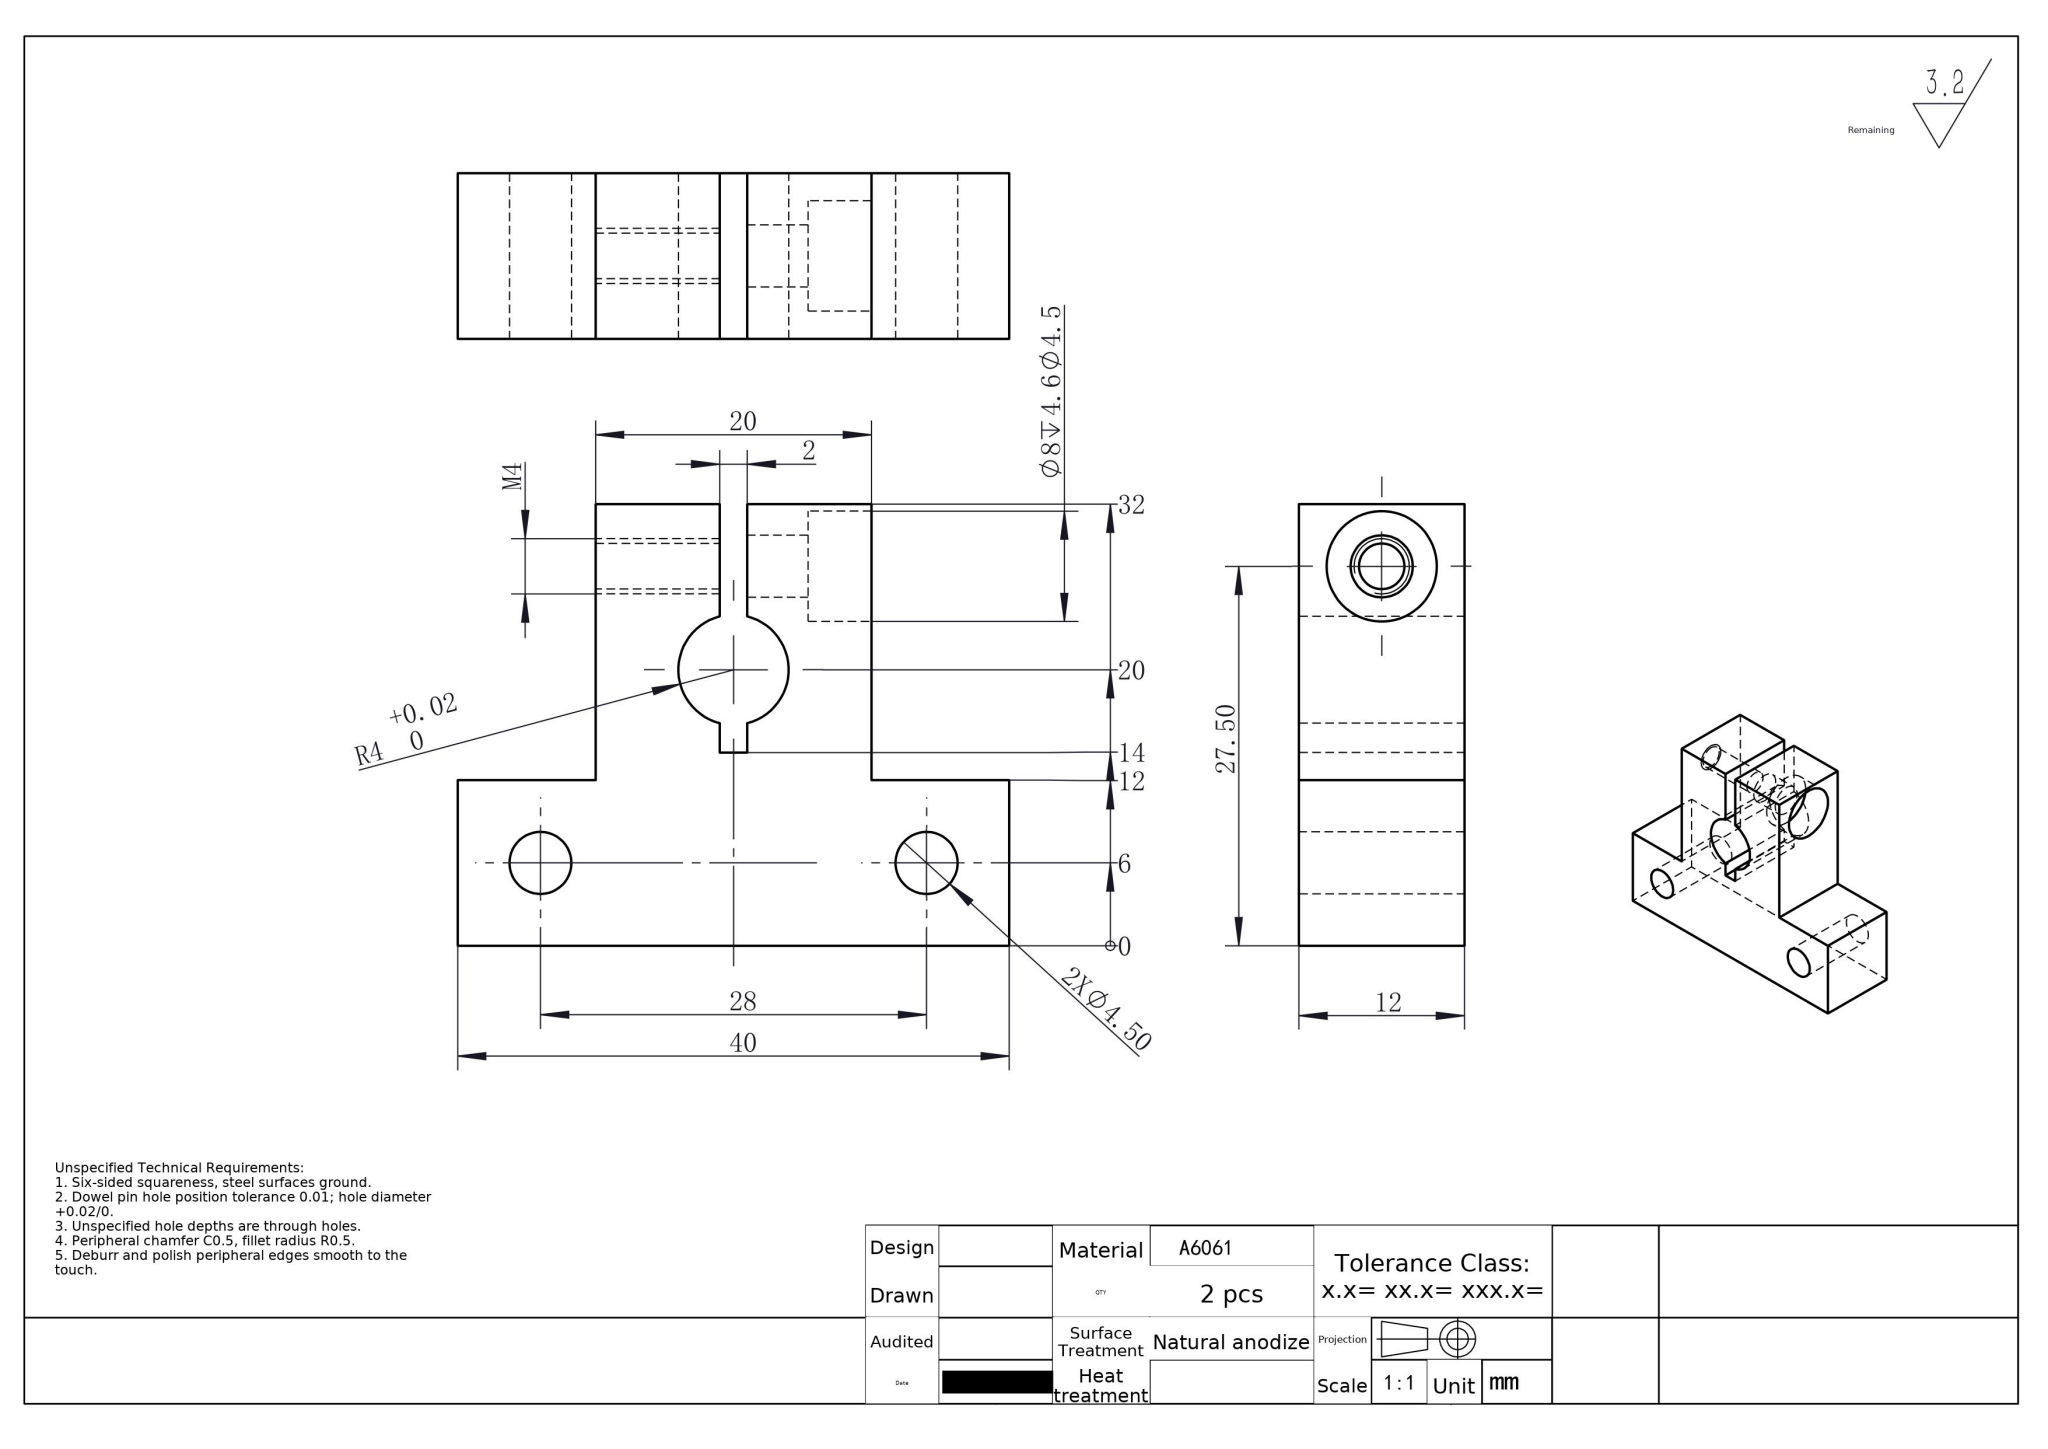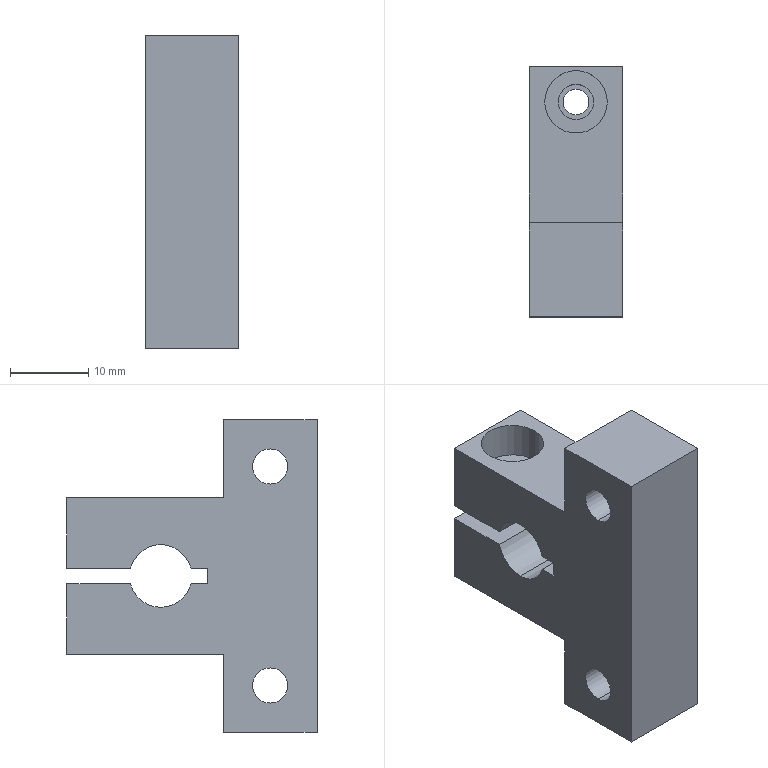Part | NX | mm | 1 solid | 30 faces | box 12 x 32 x 40 mm | volume 8955 mm3 | plane 17 | cylinder 13 | commonest cylinder face diameters 4.5 x6 8 x5 3.3 x2
STEP:
#1=CARTESIAN_POINT('',(0.,25.85,-1.));
#2=VERTEX_POINT('',#1);
#3=CARTESIAN_POINT('',(0.,29.15,-1.));
#4=VERTEX_POINT('',#3);
#5=CARTESIAN_POINT('',(0.,27.5,-1.));
#6=DIRECTION('',(0.,0.,-1.));
#7=DIRECTION('',(-1.,0.,0.));
#8=AXIS2_PLACEMENT_3D('',#5,#6,#7);
#9=CIRCLE('',#8,1.65);
#10=EDGE_CURVE('',#2,#4,#9,.T.);
#11=ORIENTED_EDGE('',*,*,#10,.F.);
#12=CARTESIAN_POINT('',(0.,25.85,-10.));
#13=VERTEX_POINT('',#12);
#14=CARTESIAN_POINT('',(0.,25.85,-10.));
#15=DIRECTION('',(0.,0.,-1.));
#16=VECTOR('',#15,1000.);
#17=LINE('',#14,#16);
#18=EDGE_CURVE('',#2,#13,#17,.T.);
#19=ORIENTED_EDGE('',*,*,#18,.T.);
#20=CARTESIAN_POINT('',(0.,29.15,-10.));
#21=VERTEX_POINT('',#20);
#22=CARTESIAN_POINT('',(0.,27.5,-10.));
#23=DIRECTION('',(0.,0.,-1.));
#24=DIRECTION('',(0.,1.,0.));
#25=AXIS2_PLACEMENT_3D('',#22,#23,#24);
#26=CIRCLE('',#25,1.65);
#27=EDGE_CURVE('',#13,#21,#26,.T.);
#28=ORIENTED_EDGE('',*,*,#27,.T.);
#29=CARTESIAN_POINT('',(0.,29.15,-10.));
#30=DIRECTION('',(0.,0.,-1.));
#31=VECTOR('',#30,1000.);
#32=LINE('',#29,#31);
#33=EDGE_CURVE('',#4,#21,#32,.T.);
#34=ORIENTED_EDGE('',*,*,#33,.F.);
#35=EDGE_LOOP('',(#11,#19,#28,#34));
#36=FACE_OUTER_BOUND('',#35,.T.);
#37=CARTESIAN_POINT('',(0.,27.5,-10.));
#38=DIRECTION('',(0.,0.,-1.));
#39=DIRECTION('',(0.,1.,0.));
#40=AXIS2_PLACEMENT_3D('',#37,#38,#39);
#41=CYLINDRICAL_SURFACE('',#40,1.65);
#42=ADVANCED_FACE('',(#36),#41,.F.);
#43=CARTESIAN_POINT('',(-4.,27.5,5.4));
#44=VERTEX_POINT('',#43);
#45=CARTESIAN_POINT('',(4.,27.5,5.4));
#46=VERTEX_POINT('',#45);
#47=CARTESIAN_POINT('',(0.,27.5,5.4));
#48=DIRECTION('',(0.,0.,1.));
#49=DIRECTION('',(1.,0.,0.));
#50=AXIS2_PLACEMENT_3D('',#47,#48,#49);
#51=CIRCLE('',#50,4.);
#52=EDGE_CURVE('',#44,#46,#51,.T.);
#53=ORIENTED_EDGE('',*,*,#52,.F.);
#54=CARTESIAN_POINT('',(-4.,27.5,10.));
#55=VERTEX_POINT('',#54);
#56=CARTESIAN_POINT('',(-4.,27.5,10.));
#57=DIRECTION('',(0.,0.,1.));
#58=VECTOR('',#57,1000.);
#59=LINE('',#56,#58);
#60=EDGE_CURVE('',#44,#55,#59,.T.);
#61=ORIENTED_EDGE('',*,*,#60,.T.);
#62=CARTESIAN_POINT('',(4.,27.5,10.));
#63=VERTEX_POINT('',#62);
#64=CARTESIAN_POINT('',(0.,27.5,10.));
#65=DIRECTION('',(0.,0.,1.));
#66=DIRECTION('',(1.,0.,0.));
#67=AXIS2_PLACEMENT_3D('',#64,#65,#66);
#68=CIRCLE('',#67,4.);
#69=EDGE_CURVE('',#55,#63,#68,.T.);
#70=ORIENTED_EDGE('',*,*,#69,.T.);
#71=CARTESIAN_POINT('',(4.,27.5,10.));
#72=DIRECTION('',(0.,0.,1.));
#73=VECTOR('',#72,1000.);
#74=LINE('',#71,#73);
#75=EDGE_CURVE('',#46,#63,#74,.T.);
#76=ORIENTED_EDGE('',*,*,#75,.F.);
#77=EDGE_LOOP('',(#53,#61,#70,#76));
#78=FACE_OUTER_BOUND('',#77,.T.);
#79=CARTESIAN_POINT('',(0.,27.5,10.));
#80=DIRECTION('',(0.,0.,1.));
#81=DIRECTION('',(1.,0.,0.));
#82=AXIS2_PLACEMENT_3D('',#79,#80,#81);
#83=CYLINDRICAL_SURFACE('',#82,4.);
#84=ADVANCED_FACE('',(#78),#83,.F.);
#85=CARTESIAN_POINT('',(-2.25,27.5,1.));
#86=VERTEX_POINT('',#85);
#87=CARTESIAN_POINT('',(2.25,27.5,1.));
#88=VERTEX_POINT('',#87);
#89=CARTESIAN_POINT('',(0.,27.5,1.));
#90=DIRECTION('',(0.,-0.,1.));
#91=DIRECTION('',(0.,-1.,-0.));
#92=AXIS2_PLACEMENT_3D('',#89,#90,#91);
#93=CIRCLE('',#92,2.25);
#94=EDGE_CURVE('',#86,#88,#93,.T.);
#95=ORIENTED_EDGE('',*,*,#94,.F.);
#96=CARTESIAN_POINT('',(-2.25,27.5,5.4));
#97=VERTEX_POINT('',#96);
#98=CARTESIAN_POINT('',(-2.25,27.5,10.));
#99=DIRECTION('',(0.,0.,1.));
#100=VECTOR('',#99,1000.);
#101=LINE('',#98,#100);
#102=EDGE_CURVE('',#86,#97,#101,.T.);
#103=ORIENTED_EDGE('',*,*,#102,.T.);
#104=CARTESIAN_POINT('',(2.25,27.5,5.4));
#105=VERTEX_POINT('',#104);
#106=CARTESIAN_POINT('',(0.,27.5,5.4));
#107=DIRECTION('',(0.,0.,1.));
#108=DIRECTION('',(1.,0.,0.));
#109=AXIS2_PLACEMENT_3D('',#106,#107,#108);
#110=CIRCLE('',#109,2.25);
#111=EDGE_CURVE('',#97,#105,#110,.T.);
#112=ORIENTED_EDGE('',*,*,#111,.T.);
#113=CARTESIAN_POINT('',(2.25,27.5,10.));
#114=DIRECTION('',(0.,0.,1.));
#115=VECTOR('',#114,1000.);
#116=LINE('',#113,#115);
#117=EDGE_CURVE('',#88,#105,#116,.T.);
#118=ORIENTED_EDGE('',*,*,#117,.F.);
#119=EDGE_LOOP('',(#95,#103,#112,#118));
#120=FACE_OUTER_BOUND('',#119,.T.);
#121=CARTESIAN_POINT('',(0.,27.5,10.));
#122=DIRECTION('',(0.,0.,1.));
#123=DIRECTION('',(1.,0.,0.));
#124=AXIS2_PLACEMENT_3D('',#121,#122,#123);
#125=CYLINDRICAL_SURFACE('',#124,2.25);
#126=ADVANCED_FACE('',(#120),#125,.F.);
#127=CARTESIAN_POINT('',(-6.,6.,-16.25));
#128=VERTEX_POINT('',#127);
#129=CARTESIAN_POINT('',(-6.,6.,-11.75));
#130=VERTEX_POINT('',#129);
#131=CARTESIAN_POINT('',(-6.,6.,-14.));
#132=DIRECTION('',(-1.,0.,0.));
#133=DIRECTION('',(0.,0.,1.));
#134=AXIS2_PLACEMENT_3D('',#131,#132,#133);
#135=CIRCLE('',#134,2.25);
#136=EDGE_CURVE('',#128,#130,#135,.T.);
#137=ORIENTED_EDGE('',*,*,#136,.T.);
#138=CARTESIAN_POINT('',(6.,6.,-11.75));
#139=VERTEX_POINT('',#138);
#140=CARTESIAN_POINT('',(-14.,6.,-11.75));
#141=DIRECTION('',(1.,0.,0.));
#142=VECTOR('',#141,1000.);
#143=LINE('',#140,#142);
#144=EDGE_CURVE('',#130,#139,#143,.T.);
#145=ORIENTED_EDGE('',*,*,#144,.T.);
#146=CARTESIAN_POINT('',(6.,6.,-16.25));
#147=VERTEX_POINT('',#146);
#148=CARTESIAN_POINT('',(6.,6.,-14.));
#149=DIRECTION('',(1.,0.,0.));
#150=DIRECTION('',(0.,0.,-1.));
#151=AXIS2_PLACEMENT_3D('',#148,#149,#150);
#152=CIRCLE('',#151,2.25);
#153=EDGE_CURVE('',#139,#147,#152,.T.);
#154=ORIENTED_EDGE('',*,*,#153,.T.);
#155=CARTESIAN_POINT('',(-14.,6.,-16.25));
#156=DIRECTION('',(1.,0.,0.));
#157=VECTOR('',#156,1000.);
#158=LINE('',#155,#157);
#159=EDGE_CURVE('',#128,#147,#158,.T.);
#160=ORIENTED_EDGE('',*,*,#159,.F.);
#161=EDGE_LOOP('',(#137,#145,#154,#160));
#162=FACE_OUTER_BOUND('',#161,.T.);
#163=CARTESIAN_POINT('',(-14.,6.,-14.));
#164=DIRECTION('',(1.,0.,0.));
#165=DIRECTION('',(0.,0.,-1.));
#166=AXIS2_PLACEMENT_3D('',#163,#164,#165);
#167=CYLINDRICAL_SURFACE('',#166,2.25);
#168=ADVANCED_FACE('',(#162),#167,.F.);
#169=CARTESIAN_POINT('',(-6.,6.,11.75));
#170=VERTEX_POINT('',#169);
#171=CARTESIAN_POINT('',(-6.,6.,16.25));
#172=VERTEX_POINT('',#171);
#173=CARTESIAN_POINT('',(-6.,6.,14.));
#174=DIRECTION('',(-1.,0.,0.));
#175=DIRECTION('',(0.,0.,1.));
#176=AXIS2_PLACEMENT_3D('',#173,#174,#175);
#177=CIRCLE('',#176,2.25);
#178=EDGE_CURVE('',#170,#172,#177,.T.);
#179=ORIENTED_EDGE('',*,*,#178,.T.);
#180=CARTESIAN_POINT('',(6.,6.,16.25));
#181=VERTEX_POINT('',#180);
#182=CARTESIAN_POINT('',(-14.,6.,16.25));
#183=DIRECTION('',(1.,0.,0.));
#184=VECTOR('',#183,1000.);
#185=LINE('',#182,#184);
#186=EDGE_CURVE('',#172,#181,#185,.T.);
#187=ORIENTED_EDGE('',*,*,#186,.T.);
#188=CARTESIAN_POINT('',(6.,6.,11.75));
#189=VERTEX_POINT('',#188);
#190=CARTESIAN_POINT('',(6.,6.,14.));
#191=DIRECTION('',(1.,0.,0.));
#192=DIRECTION('',(0.,0.,-1.));
#193=AXIS2_PLACEMENT_3D('',#190,#191,#192);
#194=CIRCLE('',#193,2.25);
#195=EDGE_CURVE('',#181,#189,#194,.T.);
#196=ORIENTED_EDGE('',*,*,#195,.T.);
#197=CARTESIAN_POINT('',(-14.,6.,11.75));
#198=DIRECTION('',(1.,0.,0.));
#199=VECTOR('',#198,1000.);
#200=LINE('',#197,#199);
#201=EDGE_CURVE('',#170,#189,#200,.T.);
#202=ORIENTED_EDGE('',*,*,#201,.F.);
#203=EDGE_LOOP('',(#179,#187,#196,#202));
#204=FACE_OUTER_BOUND('',#203,.T.);
#205=CARTESIAN_POINT('',(-14.,6.,14.));
#206=DIRECTION('',(1.,0.,0.));
#207=DIRECTION('',(0.,0.,-1.));
#208=AXIS2_PLACEMENT_3D('',#205,#206,#207);
#209=CYLINDRICAL_SURFACE('',#208,2.25);
#210=ADVANCED_FACE('',(#204),#209,.F.);
#211=CARTESIAN_POINT('',(-6.,23.873,-1.));
#212=VERTEX_POINT('',#211);
#213=CARTESIAN_POINT('',(-6.,20.,-4.));
#214=VERTEX_POINT('',#213);
#215=CARTESIAN_POINT('',(-6.,20.,0.));
#216=DIRECTION('',(-1.,0.,0.));
#217=DIRECTION('',(0.,0.,1.));
#218=AXIS2_PLACEMENT_3D('',#215,#216,#217);
#219=CIRCLE('',#218,4.);
#220=EDGE_CURVE('',#212,#214,#219,.T.);
#221=ORIENTED_EDGE('',*,*,#220,.T.);
#222=CARTESIAN_POINT('',(6.,20.,-4.));
#223=VERTEX_POINT('',#222);
#224=CARTESIAN_POINT('',(-31.,20.,-4.));
#225=DIRECTION('',(1.,0.,0.));
#226=VECTOR('',#225,1000.);
#227=LINE('',#224,#226);
#228=EDGE_CURVE('',#214,#223,#227,.T.);
#229=ORIENTED_EDGE('',*,*,#228,.T.);
#230=CARTESIAN_POINT('',(6.,23.873,-1.));
#231=VERTEX_POINT('',#230);
#232=CARTESIAN_POINT('',(6.,20.,0.));
#233=DIRECTION('',(-1.,0.,0.));
#234=DIRECTION('',(0.,0.,1.));
#235=AXIS2_PLACEMENT_3D('',#232,#233,#234);
#236=CIRCLE('',#235,4.);
#237=EDGE_CURVE('',#231,#223,#236,.T.);
#238=ORIENTED_EDGE('',*,*,#237,.F.);
#239=CARTESIAN_POINT('',(-31.,23.873,-1.));
#240=DIRECTION('',(1.,0.,0.));
#241=VECTOR('',#240,1000.);
#242=LINE('',#239,#241);
#243=EDGE_CURVE('',#212,#231,#242,.T.);
#244=ORIENTED_EDGE('',*,*,#243,.F.);
#245=EDGE_LOOP('',(#221,#229,#238,#244));
#246=FACE_OUTER_BOUND('',#245,.T.);
#247=CARTESIAN_POINT('',(-31.,20.,0.));
#248=DIRECTION('',(1.,0.,0.));
#249=DIRECTION('',(0.,0.,-1.));
#250=AXIS2_PLACEMENT_3D('',#247,#248,#249);
#251=CYLINDRICAL_SURFACE('',#250,4.);
#252=ADVANCED_FACE('',(#246),#251,.F.);
#253=CARTESIAN_POINT('',(-6.,32.,-10.));
#254=VERTEX_POINT('',#253);
#255=CARTESIAN_POINT('',(-6.,32.,-1.));
#256=VERTEX_POINT('',#255);
#257=CARTESIAN_POINT('',(-6.,32.,10.));
#258=DIRECTION('',(0.,0.,1.));
#259=VECTOR('',#258,1000.);
#260=LINE('',#257,#259);
#261=EDGE_CURVE('',#254,#256,#260,.T.);
#262=ORIENTED_EDGE('',*,*,#261,.T.);
#263=CARTESIAN_POINT('',(6.,32.,-1.));
#264=VERTEX_POINT('',#263);
#265=CARTESIAN_POINT('',(-31.,32.,-1.));
#266=DIRECTION('',(1.,0.,0.));
#267=VECTOR('',#266,1000.);
#268=LINE('',#265,#267);
#269=EDGE_CURVE('',#256,#264,#268,.T.);
#270=ORIENTED_EDGE('',*,*,#269,.T.);
#271=CARTESIAN_POINT('',(6.,32.,-10.));
#272=VERTEX_POINT('',#271);
#273=CARTESIAN_POINT('',(6.,32.,10.));
#274=DIRECTION('',(0.,0.,1.));
#275=VECTOR('',#274,1000.);
#276=LINE('',#273,#275);
#277=EDGE_CURVE('',#272,#264,#276,.T.);
#278=ORIENTED_EDGE('',*,*,#277,.F.);
#279=CARTESIAN_POINT('',(6.,32.,-10.));
#280=DIRECTION('',(-1.,0.,0.));
#281=VECTOR('',#280,1000.);
#282=LINE('',#279,#281);
#283=EDGE_CURVE('',#272,#254,#282,.T.);
#284=ORIENTED_EDGE('',*,*,#283,.T.);
#285=EDGE_LOOP('',(#262,#270,#278,#284));
#286=FACE_OUTER_BOUND('',#285,.T.);
#287=CARTESIAN_POINT('',(6.,32.,10.));
#288=DIRECTION('',(0.,-1.,0.));
#289=DIRECTION('',(0.,0.,-1.));
#290=AXIS2_PLACEMENT_3D('',#287,#288,#289);
#291=PLANE('',#290);
#292=ADVANCED_FACE('',(#286),#291,.F.);
#293=CARTESIAN_POINT('',(-6.,12.,20.));
#294=VERTEX_POINT('',#293);
#295=CARTESIAN_POINT('',(-6.,0.,20.));
#296=VERTEX_POINT('',#295);
#297=CARTESIAN_POINT('',(-6.,0.,20.));
#298=DIRECTION('',(0.,-1.,0.));
#299=VECTOR('',#298,1000.);
#300=LINE('',#297,#299);
#301=EDGE_CURVE('',#294,#296,#300,.T.);
#302=ORIENTED_EDGE('',*,*,#301,.T.);
#303=CARTESIAN_POINT('',(6.,0.,20.));
#304=VERTEX_POINT('',#303);
#305=CARTESIAN_POINT('',(6.,0.,20.));
#306=DIRECTION('',(-1.,0.,0.));
#307=VECTOR('',#306,1000.);
#308=LINE('',#305,#307);
#309=EDGE_CURVE('',#304,#296,#308,.T.);
#310=ORIENTED_EDGE('',*,*,#309,.F.);
#311=CARTESIAN_POINT('',(6.,12.,20.));
#312=VERTEX_POINT('',#311);
#313=CARTESIAN_POINT('',(6.,0.,20.));
#314=DIRECTION('',(0.,-1.,0.));
#315=VECTOR('',#314,1000.);
#316=LINE('',#313,#315);
#317=EDGE_CURVE('',#312,#304,#316,.T.);
#318=ORIENTED_EDGE('',*,*,#317,.F.);
#319=CARTESIAN_POINT('',(6.,12.,20.));
#320=DIRECTION('',(-1.,0.,0.));
#321=VECTOR('',#320,1000.);
#322=LINE('',#319,#321);
#323=EDGE_CURVE('',#312,#294,#322,.T.);
#324=ORIENTED_EDGE('',*,*,#323,.T.);
#325=EDGE_LOOP('',(#302,#310,#318,#324));
#326=FACE_OUTER_BOUND('',#325,.T.);
#327=CARTESIAN_POINT('',(6.,0.,20.));
#328=DIRECTION('',(0.,-0.,-1.));
#329=DIRECTION('',(0.,1.,-0.));
#330=AXIS2_PLACEMENT_3D('',#327,#328,#329);
#331=PLANE('',#330);
#332=ADVANCED_FACE('',(#326),#331,.F.);
#333=CARTESIAN_POINT('',(-6.,0.,-20.));
#334=VERTEX_POINT('',#333);
#335=CARTESIAN_POINT('',(-6.,0.,20.));
#336=DIRECTION('',(0.,0.,-1.));
#337=VECTOR('',#336,1000.);
#338=LINE('',#335,#337);
#339=EDGE_CURVE('',#296,#334,#338,.T.);
#340=ORIENTED_EDGE('',*,*,#339,.T.);
#341=CARTESIAN_POINT('',(6.,0.,-20.));
#342=VERTEX_POINT('',#341);
#343=CARTESIAN_POINT('',(6.,0.,-20.));
#344=DIRECTION('',(-1.,0.,0.));
#345=VECTOR('',#344,1000.);
#346=LINE('',#343,#345);
#347=EDGE_CURVE('',#342,#334,#346,.T.);
#348=ORIENTED_EDGE('',*,*,#347,.F.);
#349=CARTESIAN_POINT('',(6.,0.,20.));
#350=DIRECTION('',(0.,0.,-1.));
#351=VECTOR('',#350,1000.);
#352=LINE('',#349,#351);
#353=EDGE_CURVE('',#304,#342,#352,.T.);
#354=ORIENTED_EDGE('',*,*,#353,.F.);
#355=ORIENTED_EDGE('',*,*,#309,.T.);
#356=EDGE_LOOP('',(#340,#348,#354,#355));
#357=FACE_OUTER_BOUND('',#356,.T.);
#358=CARTESIAN_POINT('',(6.,0.,20.));
#359=DIRECTION('',(0.,1.,0.));
#360=DIRECTION('',(0.,0.,1.));
#361=AXIS2_PLACEMENT_3D('',#358,#359,#360);
#362=PLANE('',#361);
#363=ADVANCED_FACE('',(#357),#362,.F.);
#364=CARTESIAN_POINT('',(-6.,12.,-20.));
#365=VERTEX_POINT('',#364);
#366=CARTESIAN_POINT('',(-6.,12.,-20.));
#367=DIRECTION('',(0.,1.,0.));
#368=VECTOR('',#367,1000.);
#369=LINE('',#366,#368);
#370=EDGE_CURVE('',#334,#365,#369,.T.);
#371=ORIENTED_EDGE('',*,*,#370,.T.);
#372=CARTESIAN_POINT('',(6.,12.,-20.));
#373=VERTEX_POINT('',#372);
#374=CARTESIAN_POINT('',(6.,12.,-20.));
#375=DIRECTION('',(-1.,0.,0.));
#376=VECTOR('',#375,1000.);
#377=LINE('',#374,#376);
#378=EDGE_CURVE('',#373,#365,#377,.T.);
#379=ORIENTED_EDGE('',*,*,#378,.F.);
#380=CARTESIAN_POINT('',(6.,12.,-20.));
#381=DIRECTION('',(0.,1.,0.));
#382=VECTOR('',#381,1000.);
#383=LINE('',#380,#382);
#384=EDGE_CURVE('',#342,#373,#383,.T.);
#385=ORIENTED_EDGE('',*,*,#384,.F.);
#386=ORIENTED_EDGE('',*,*,#347,.T.);
#387=EDGE_LOOP('',(#371,#379,#385,#386));
#388=FACE_OUTER_BOUND('',#387,.T.);
#389=CARTESIAN_POINT('',(6.,12.,-20.));
#390=DIRECTION('',(0.,-0.,1.));
#391=DIRECTION('',(0.,-1.,-0.));
#392=AXIS2_PLACEMENT_3D('',#389,#390,#391);
#393=PLANE('',#392);
#394=ADVANCED_FACE('',(#388),#393,.F.);
#395=CARTESIAN_POINT('',(-6.,12.,-10.));
#396=VERTEX_POINT('',#395);
#397=CARTESIAN_POINT('',(-6.,12.,-10.));
#398=DIRECTION('',(0.,0.,1.));
#399=VECTOR('',#398,1000.);
#400=LINE('',#397,#399);
#401=EDGE_CURVE('',#365,#396,#400,.T.);
#402=ORIENTED_EDGE('',*,*,#401,.T.);
#403=CARTESIAN_POINT('',(6.,12.,-10.));
#404=VERTEX_POINT('',#403);
#405=CARTESIAN_POINT('',(6.,12.,-10.));
#406=DIRECTION('',(-1.,0.,0.));
#407=VECTOR('',#406,1000.);
#408=LINE('',#405,#407);
#409=EDGE_CURVE('',#404,#396,#408,.T.);
#410=ORIENTED_EDGE('',*,*,#409,.F.);
#411=CARTESIAN_POINT('',(6.,12.,-10.));
#412=DIRECTION('',(0.,0.,1.));
#413=VECTOR('',#412,1000.);
#414=LINE('',#411,#413);
#415=EDGE_CURVE('',#373,#404,#414,.T.);
#416=ORIENTED_EDGE('',*,*,#415,.F.);
#417=ORIENTED_EDGE('',*,*,#378,.T.);
#418=EDGE_LOOP('',(#402,#410,#416,#417));
#419=FACE_OUTER_BOUND('',#418,.T.);
#420=CARTESIAN_POINT('',(6.,12.,-10.));
#421=DIRECTION('',(0.,-1.,0.));
#422=DIRECTION('',(0.,0.,-1.));
#423=AXIS2_PLACEMENT_3D('',#420,#421,#422);
#424=PLANE('',#423);
#425=ADVANCED_FACE('',(#419),#424,.F.);
#426=CARTESIAN_POINT('',(0.,27.5,-10.));
#427=DIRECTION('',(0.,0.,-1.));
#428=DIRECTION('',(0.,1.,0.));
#429=AXIS2_PLACEMENT_3D('',#426,#427,#428);
#430=CIRCLE('',#429,1.65);
#431=EDGE_CURVE('',#21,#13,#430,.T.);
#432=ORIENTED_EDGE('',*,*,#431,.F.);
#433=ORIENTED_EDGE('',*,*,#27,.F.);
#434=EDGE_LOOP('',(#432,#433));
#435=FACE_BOUND('',#434,.T.);
#436=CARTESIAN_POINT('',(-6.,32.,-10.));
#437=DIRECTION('',(0.,1.,0.));
#438=VECTOR('',#437,1000.);
#439=LINE('',#436,#438);
#440=EDGE_CURVE('',#396,#254,#439,.T.);
#441=ORIENTED_EDGE('',*,*,#440,.T.);
#442=ORIENTED_EDGE('',*,*,#283,.F.);
#443=CARTESIAN_POINT('',(6.,32.,-10.));
#444=DIRECTION('',(0.,1.,0.));
#445=VECTOR('',#444,1000.);
#446=LINE('',#443,#445);
#447=EDGE_CURVE('',#404,#272,#446,.T.);
#448=ORIENTED_EDGE('',*,*,#447,.F.);
#449=ORIENTED_EDGE('',*,*,#409,.T.);
#450=EDGE_LOOP('',(#441,#442,#448,#449));
#451=FACE_OUTER_BOUND('',#450,.T.);
#452=CARTESIAN_POINT('',(6.,32.,-10.));
#453=DIRECTION('',(0.,-0.,1.));
#454=DIRECTION('',(0.,-1.,-0.));
#455=AXIS2_PLACEMENT_3D('',#452,#453,#454);
#456=PLANE('',#455);
#457=ADVANCED_FACE('',(#435,#451),#456,.F.);
#458=CARTESIAN_POINT('',(6.,32.,1.));
#459=VERTEX_POINT('',#458);
#460=CARTESIAN_POINT('',(6.,32.,10.));
#461=VERTEX_POINT('',#460);
#462=CARTESIAN_POINT('',(6.,32.,10.));
#463=DIRECTION('',(0.,0.,1.));
#464=VECTOR('',#463,1000.);
#465=LINE('',#462,#464);
#466=EDGE_CURVE('',#459,#461,#465,.T.);
#467=ORIENTED_EDGE('',*,*,#466,.F.);
#468=CARTESIAN_POINT('',(-6.,32.,1.));
#469=VERTEX_POINT('',#468);
#470=CARTESIAN_POINT('',(-31.,32.,1.));
#471=DIRECTION('',(1.,0.,0.));
#472=VECTOR('',#471,1000.);
#473=LINE('',#470,#472);
#474=EDGE_CURVE('',#469,#459,#473,.T.);
#475=ORIENTED_EDGE('',*,*,#474,.F.);
#476=CARTESIAN_POINT('',(-6.,32.,10.));
#477=VERTEX_POINT('',#476);
#478=CARTESIAN_POINT('',(-6.,32.,10.));
#479=DIRECTION('',(0.,0.,1.));
#480=VECTOR('',#479,1000.);
#481=LINE('',#478,#480);
#482=EDGE_CURVE('',#469,#477,#481,.T.);
#483=ORIENTED_EDGE('',*,*,#482,.T.);
#484=CARTESIAN_POINT('',(6.,32.,10.));
#485=DIRECTION('',(-1.,0.,0.));
#486=VECTOR('',#485,1000.);
#487=LINE('',#484,#486);
#488=EDGE_CURVE('',#461,#477,#487,.T.);
#489=ORIENTED_EDGE('',*,*,#488,.F.);
#490=EDGE_LOOP('',(#467,#475,#483,#489));
#491=FACE_OUTER_BOUND('',#490,.T.);
#492=CARTESIAN_POINT('',(6.,32.,10.));
#493=DIRECTION('',(0.,-1.,0.));
#494=DIRECTION('',(0.,0.,-1.));
#495=AXIS2_PLACEMENT_3D('',#492,#493,#494);
#496=PLANE('',#495);
#497=ADVANCED_FACE('',(#491),#496,.F.);
#498=CARTESIAN_POINT('',(0.,27.5,10.));
#499=DIRECTION('',(0.,0.,1.));
#500=DIRECTION('',(1.,0.,0.));
#501=AXIS2_PLACEMENT_3D('',#498,#499,#500);
#502=CIRCLE('',#501,4.);
#503=EDGE_CURVE('',#63,#55,#502,.T.);
#504=ORIENTED_EDGE('',*,*,#503,.F.);
#505=ORIENTED_EDGE('',*,*,#69,.F.);
#506=EDGE_LOOP('',(#504,#505));
#507=FACE_BOUND('',#506,.T.);
#508=CARTESIAN_POINT('',(-6.,12.,10.));
#509=VERTEX_POINT('',#508);
#510=CARTESIAN_POINT('',(-6.,12.,10.));
#511=DIRECTION('',(0.,-1.,0.));
#512=VECTOR('',#511,1000.);
#513=LINE('',#510,#512);
#514=EDGE_CURVE('',#477,#509,#513,.T.);
#515=ORIENTED_EDGE('',*,*,#514,.T.);
#516=CARTESIAN_POINT('',(6.,12.,10.));
#517=VERTEX_POINT('',#516);
#518=CARTESIAN_POINT('',(6.,12.,10.));
#519=DIRECTION('',(-1.,0.,0.));
#520=VECTOR('',#519,1000.);
#521=LINE('',#518,#520);
#522=EDGE_CURVE('',#517,#509,#521,.T.);
#523=ORIENTED_EDGE('',*,*,#522,.F.);
#524=CARTESIAN_POINT('',(6.,12.,10.));
#525=DIRECTION('',(0.,-1.,0.));
#526=VECTOR('',#525,1000.);
#527=LINE('',#524,#526);
#528=EDGE_CURVE('',#461,#517,#527,.T.);
#529=ORIENTED_EDGE('',*,*,#528,.F.);
#530=ORIENTED_EDGE('',*,*,#488,.T.);
#531=EDGE_LOOP('',(#515,#523,#529,#530));
#532=FACE_OUTER_BOUND('',#531,.T.);
#533=CARTESIAN_POINT('',(6.,12.,10.));
#534=DIRECTION('',(0.,0.,-1.));
#535=DIRECTION('',(-1.,0.,0.));
#536=AXIS2_PLACEMENT_3D('',#533,#534,#535);
#537=PLANE('',#536);
#538=ADVANCED_FACE('',(#507,#532),#537,.F.);
#539=CARTESIAN_POINT('',(-6.,12.,20.));
#540=DIRECTION('',(0.,0.,1.));
#541=VECTOR('',#540,1000.);
#542=LINE('',#539,#541);
#543=EDGE_CURVE('',#509,#294,#542,.T.);
#544=ORIENTED_EDGE('',*,*,#543,.T.);
#545=ORIENTED_EDGE('',*,*,#323,.F.);
#546=CARTESIAN_POINT('',(6.,12.,20.));
#547=DIRECTION('',(0.,0.,1.));
#548=VECTOR('',#547,1000.);
#549=LINE('',#546,#548);
#550=EDGE_CURVE('',#517,#312,#549,.T.);
#551=ORIENTED_EDGE('',*,*,#550,.F.);
#552=ORIENTED_EDGE('',*,*,#522,.T.);
#553=EDGE_LOOP('',(#544,#545,#551,#552));
#554=FACE_OUTER_BOUND('',#553,.T.);
#555=CARTESIAN_POINT('',(6.,12.,20.));
#556=DIRECTION('',(0.,-1.,0.));
#557=DIRECTION('',(0.,0.,-1.));
#558=AXIS2_PLACEMENT_3D('',#555,#556,#557);
#559=PLANE('',#558);
#560=ADVANCED_FACE('',(#554),#559,.F.);
#561=CARTESIAN_POINT('',(6.,6.,-14.));
#562=DIRECTION('',(1.,0.,0.));
#563=DIRECTION('',(0.,0.,-1.));
#564=AXIS2_PLACEMENT_3D('',#561,#562,#563);
#565=CIRCLE('',#564,2.25);
#566=EDGE_CURVE('',#147,#139,#565,.T.);
#567=ORIENTED_EDGE('',*,*,#566,.F.);
#568=ORIENTED_EDGE('',*,*,#153,.F.);
#569=EDGE_LOOP('',(#567,#568));
#570=FACE_BOUND('',#569,.T.);
#571=CARTESIAN_POINT('',(6.,6.,14.));
#572=DIRECTION('',(1.,0.,0.));
#573=DIRECTION('',(0.,0.,-1.));
#574=AXIS2_PLACEMENT_3D('',#571,#572,#573);
#575=CIRCLE('',#574,2.25);
#576=EDGE_CURVE('',#189,#181,#575,.T.);
#577=ORIENTED_EDGE('',*,*,#576,.F.);
#578=ORIENTED_EDGE('',*,*,#195,.F.);
#579=EDGE_LOOP('',(#577,#578));
#580=FACE_BOUND('',#579,.T.);
#581=ORIENTED_EDGE('',*,*,#277,.T.);
#582=CARTESIAN_POINT('',(6.,0.,-1.));
#583=DIRECTION('',(0.,-1.,0.));
#584=VECTOR('',#583,1000.);
#585=LINE('',#582,#584);
#586=EDGE_CURVE('',#264,#231,#585,.T.);
#587=ORIENTED_EDGE('',*,*,#586,.T.);
#588=ORIENTED_EDGE('',*,*,#237,.T.);
#589=CARTESIAN_POINT('',(6.,16.127,-1.));
#590=VERTEX_POINT('',#589);
#591=CARTESIAN_POINT('',(6.,20.,0.));
#592=DIRECTION('',(-1.,0.,0.));
#593=DIRECTION('',(0.,0.,1.));
#594=AXIS2_PLACEMENT_3D('',#591,#592,#593);
#595=CIRCLE('',#594,4.);
#596=EDGE_CURVE('',#223,#590,#595,.T.);
#597=ORIENTED_EDGE('',*,*,#596,.T.);
#598=CARTESIAN_POINT('',(6.,14.,-1.));
#599=VERTEX_POINT('',#598);
#600=CARTESIAN_POINT('',(6.,0.,-1.));
#601=DIRECTION('',(0.,-1.,0.));
#602=VECTOR('',#601,1000.);
#603=LINE('',#600,#602);
#604=EDGE_CURVE('',#590,#599,#603,.T.);
#605=ORIENTED_EDGE('',*,*,#604,.T.);
#606=CARTESIAN_POINT('',(6.,14.,1.));
#607=VERTEX_POINT('',#606);
#608=CARTESIAN_POINT('',(6.,14.,0.));
#609=DIRECTION('',(0.,0.,1.));
#610=VECTOR('',#609,1000.);
#611=LINE('',#608,#610);
#612=EDGE_CURVE('',#599,#607,#611,.T.);
#613=ORIENTED_EDGE('',*,*,#612,.T.);
#614=CARTESIAN_POINT('',(6.,16.127,1.));
#615=VERTEX_POINT('',#614);
#616=CARTESIAN_POINT('',(6.,0.,1.));
#617=DIRECTION('',(0.,1.,-0.));
#618=VECTOR('',#617,1000.);
#619=LINE('',#616,#618);
#620=EDGE_CURVE('',#607,#615,#619,.T.);
#621=ORIENTED_EDGE('',*,*,#620,.T.);
#622=CARTESIAN_POINT('',(6.,23.873,1.));
#623=VERTEX_POINT('',#622);
#624=CARTESIAN_POINT('',(6.,20.,0.));
#625=DIRECTION('',(-1.,0.,0.));
#626=DIRECTION('',(0.,0.,1.));
#627=AXIS2_PLACEMENT_3D('',#624,#625,#626);
#628=CIRCLE('',#627,4.);
#629=EDGE_CURVE('',#615,#623,#628,.T.);
#630=ORIENTED_EDGE('',*,*,#629,.T.);
#631=CARTESIAN_POINT('',(6.,-0.,1.));
#632=DIRECTION('',(0.,1.,0.));
#633=VECTOR('',#632,1000.);
#634=LINE('',#631,#633);
#635=EDGE_CURVE('',#623,#459,#634,.T.);
#636=ORIENTED_EDGE('',*,*,#635,.T.);
#637=ORIENTED_EDGE('',*,*,#466,.T.);
#638=ORIENTED_EDGE('',*,*,#528,.T.);
#639=ORIENTED_EDGE('',*,*,#550,.T.);
#640=ORIENTED_EDGE('',*,*,#317,.T.);
#641=ORIENTED_EDGE('',*,*,#353,.T.);
#642=ORIENTED_EDGE('',*,*,#384,.T.);
#643=ORIENTED_EDGE('',*,*,#415,.T.);
#644=ORIENTED_EDGE('',*,*,#447,.T.);
#645=EDGE_LOOP('',(#581,#587,#588,#597,#605,#613,#621,#630,#636,#637,#638,#639,#640,#641,#642,#643,#644));
#646=FACE_OUTER_BOUND('',#645,.T.);
#647=CARTESIAN_POINT('',(6.,0.,0.));
#648=DIRECTION('',(-1.,0.,0.));
#649=DIRECTION('',(0.,0.,1.));
#650=AXIS2_PLACEMENT_3D('',#647,#648,#649);
#651=PLANE('',#650);
#652=ADVANCED_FACE('',(#570,#580,#646),#651,.F.);
#653=ORIENTED_EDGE('',*,*,#136,.F.);
#654=CARTESIAN_POINT('',(-6.,6.,-14.));
#655=DIRECTION('',(-1.,0.,0.));
#656=DIRECTION('',(0.,0.,1.));
#657=AXIS2_PLACEMENT_3D('',#654,#655,#656);
#658=CIRCLE('',#657,2.25);
#659=EDGE_CURVE('',#130,#128,#658,.T.);
#660=ORIENTED_EDGE('',*,*,#659,.F.);
#661=EDGE_LOOP('',(#653,#660));
#662=FACE_BOUND('',#661,.T.);
#663=ORIENTED_EDGE('',*,*,#178,.F.);
#664=CARTESIAN_POINT('',(-6.,6.,14.));
#665=DIRECTION('',(-1.,0.,0.));
#666=DIRECTION('',(0.,0.,1.));
#667=AXIS2_PLACEMENT_3D('',#664,#665,#666);
#668=CIRCLE('',#667,2.25);
#669=EDGE_CURVE('',#172,#170,#668,.T.);
#670=ORIENTED_EDGE('',*,*,#669,.F.);
#671=EDGE_LOOP('',(#663,#670));
#672=FACE_BOUND('',#671,.T.);
#673=CARTESIAN_POINT('',(-6.,0.,-1.));
#674=DIRECTION('',(0.,-1.,0.));
#675=VECTOR('',#674,1000.);
#676=LINE('',#673,#675);
#677=EDGE_CURVE('',#256,#212,#676,.T.);
#678=ORIENTED_EDGE('',*,*,#677,.F.);
#679=ORIENTED_EDGE('',*,*,#261,.F.);
#680=ORIENTED_EDGE('',*,*,#440,.F.);
#681=ORIENTED_EDGE('',*,*,#401,.F.);
#682=ORIENTED_EDGE('',*,*,#370,.F.);
#683=ORIENTED_EDGE('',*,*,#339,.F.);
#684=ORIENTED_EDGE('',*,*,#301,.F.);
#685=ORIENTED_EDGE('',*,*,#543,.F.);
#686=ORIENTED_EDGE('',*,*,#514,.F.);
#687=ORIENTED_EDGE('',*,*,#482,.F.);
#688=CARTESIAN_POINT('',(-6.,23.873,1.));
#689=VERTEX_POINT('',#688);
#690=CARTESIAN_POINT('',(-6.,-0.,1.));
#691=DIRECTION('',(0.,1.,0.));
#692=VECTOR('',#691,1000.);
#693=LINE('',#690,#692);
#694=EDGE_CURVE('',#689,#469,#693,.T.);
#695=ORIENTED_EDGE('',*,*,#694,.F.);
#696=CARTESIAN_POINT('',(-6.,16.127,1.));
#697=VERTEX_POINT('',#696);
#698=CARTESIAN_POINT('',(-6.,20.,0.));
#699=DIRECTION('',(-1.,0.,0.));
#700=DIRECTION('',(0.,0.,1.));
#701=AXIS2_PLACEMENT_3D('',#698,#699,#700);
#702=CIRCLE('',#701,4.);
#703=EDGE_CURVE('',#697,#689,#702,.T.);
#704=ORIENTED_EDGE('',*,*,#703,.F.);
#705=CARTESIAN_POINT('',(-6.,14.,1.));
#706=VERTEX_POINT('',#705);
#707=CARTESIAN_POINT('',(-6.,0.,1.));
#708=DIRECTION('',(0.,1.,-0.));
#709=VECTOR('',#708,1000.);
#710=LINE('',#707,#709);
#711=EDGE_CURVE('',#706,#697,#710,.T.);
#712=ORIENTED_EDGE('',*,*,#711,.F.);
#713=CARTESIAN_POINT('',(-6.,14.,-1.));
#714=VERTEX_POINT('',#713);
#715=CARTESIAN_POINT('',(-6.,14.,0.));
#716=DIRECTION('',(0.,0.,1.));
#717=VECTOR('',#716,1000.);
#718=LINE('',#715,#717);
#719=EDGE_CURVE('',#714,#706,#718,.T.);
#720=ORIENTED_EDGE('',*,*,#719,.F.);
#721=CARTESIAN_POINT('',(-6.,16.127,-1.));
#722=VERTEX_POINT('',#721);
#723=CARTESIAN_POINT('',(-6.,0.,-1.));
#724=DIRECTION('',(0.,-1.,0.));
#725=VECTOR('',#724,1000.);
#726=LINE('',#723,#725);
#727=EDGE_CURVE('',#722,#714,#726,.T.);
#728=ORIENTED_EDGE('',*,*,#727,.F.);
#729=CARTESIAN_POINT('',(-6.,20.,0.));
#730=DIRECTION('',(-1.,0.,0.));
#731=DIRECTION('',(0.,0.,1.));
#732=AXIS2_PLACEMENT_3D('',#729,#730,#731);
#733=CIRCLE('',#732,4.);
#734=EDGE_CURVE('',#214,#722,#733,.T.);
#735=ORIENTED_EDGE('',*,*,#734,.F.);
#736=ORIENTED_EDGE('',*,*,#220,.F.);
#737=EDGE_LOOP('',(#678,#679,#680,#681,#682,#683,#684,#685,#686,#687,#695,#704,#712,#720,#728,#735,#736));
#738=FACE_OUTER_BOUND('',#737,.T.);
#739=CARTESIAN_POINT('',(-6.,0.,0.));
#740=DIRECTION('',(-1.,0.,0.));
#741=DIRECTION('',(0.,0.,1.));
#742=AXIS2_PLACEMENT_3D('',#739,#740,#741);
#743=PLANE('',#742);
#744=ADVANCED_FACE('',(#662,#672,#738),#743,.T.);
#745=CARTESIAN_POINT('',(0.,27.5,-1.));
#746=DIRECTION('',(0.,0.,-1.));
#747=DIRECTION('',(-1.,0.,0.));
#748=AXIS2_PLACEMENT_3D('',#745,#746,#747);
#749=CIRCLE('',#748,1.65);
#750=EDGE_CURVE('',#4,#2,#749,.T.);
#751=ORIENTED_EDGE('',*,*,#750,.T.);
#752=ORIENTED_EDGE('',*,*,#10,.T.);
#753=EDGE_LOOP('',(#751,#752));
#754=FACE_BOUND('',#753,.T.);
#755=ORIENTED_EDGE('',*,*,#269,.F.);
#756=ORIENTED_EDGE('',*,*,#677,.T.);
#757=ORIENTED_EDGE('',*,*,#243,.T.);
#758=ORIENTED_EDGE('',*,*,#586,.F.);
#759=EDGE_LOOP('',(#755,#756,#757,#758));
#760=FACE_OUTER_BOUND('',#759,.T.);
#761=CARTESIAN_POINT('',(-31.,23.873,-1.));
#762=DIRECTION('',(0.,0.,-1.));
#763=DIRECTION('',(-1.,0.,0.));
#764=AXIS2_PLACEMENT_3D('',#761,#762,#763);
#765=PLANE('',#764);
#766=ADVANCED_FACE('',(#754,#760),#765,.F.);
#767=ORIENTED_EDGE('',*,*,#228,.F.);
#768=ORIENTED_EDGE('',*,*,#734,.T.);
#769=CARTESIAN_POINT('',(-31.,16.127,-1.));
#770=DIRECTION('',(1.,0.,0.));
#771=VECTOR('',#770,1000.);
#772=LINE('',#769,#771);
#773=EDGE_CURVE('',#722,#590,#772,.T.);
#774=ORIENTED_EDGE('',*,*,#773,.T.);
#775=ORIENTED_EDGE('',*,*,#596,.F.);
#776=EDGE_LOOP('',(#767,#768,#774,#775));
#777=FACE_OUTER_BOUND('',#776,.T.);
#778=CARTESIAN_POINT('',(-31.,20.,0.));
#779=DIRECTION('',(1.,0.,0.));
#780=DIRECTION('',(0.,0.,-1.));
#781=AXIS2_PLACEMENT_3D('',#778,#779,#780);
#782=CYLINDRICAL_SURFACE('',#781,4.);
#783=ADVANCED_FACE('',(#777),#782,.F.);
#784=ORIENTED_EDGE('',*,*,#773,.F.);
#785=ORIENTED_EDGE('',*,*,#727,.T.);
#786=CARTESIAN_POINT('',(-31.,14.,-1.));
#787=DIRECTION('',(1.,0.,0.));
#788=VECTOR('',#787,1000.);
#789=LINE('',#786,#788);
#790=EDGE_CURVE('',#714,#599,#789,.T.);
#791=ORIENTED_EDGE('',*,*,#790,.T.);
#792=ORIENTED_EDGE('',*,*,#604,.F.);
#793=EDGE_LOOP('',(#784,#785,#791,#792));
#794=FACE_OUTER_BOUND('',#793,.T.);
#795=CARTESIAN_POINT('',(-31.,14.,-1.));
#796=DIRECTION('',(0.,0.,-1.));
#797=DIRECTION('',(-1.,0.,0.));
#798=AXIS2_PLACEMENT_3D('',#795,#796,#797);
#799=PLANE('',#798);
#800=ADVANCED_FACE('',(#794),#799,.F.);
#801=ORIENTED_EDGE('',*,*,#790,.F.);
#802=ORIENTED_EDGE('',*,*,#719,.T.);
#803=CARTESIAN_POINT('',(-31.,14.,1.));
#804=DIRECTION('',(1.,0.,0.));
#805=VECTOR('',#804,1000.);
#806=LINE('',#803,#805);
#807=EDGE_CURVE('',#706,#607,#806,.T.);
#808=ORIENTED_EDGE('',*,*,#807,.T.);
#809=ORIENTED_EDGE('',*,*,#612,.F.);
#810=EDGE_LOOP('',(#801,#802,#808,#809));
#811=FACE_OUTER_BOUND('',#810,.T.);
#812=CARTESIAN_POINT('',(-31.,14.,1.));
#813=DIRECTION('',(0.,-1.,0.));
#814=DIRECTION('',(0.,0.,-1.));
#815=AXIS2_PLACEMENT_3D('',#812,#813,#814);
#816=PLANE('',#815);
#817=ADVANCED_FACE('',(#811),#816,.F.);
#818=ORIENTED_EDGE('',*,*,#807,.F.);
#819=ORIENTED_EDGE('',*,*,#711,.T.);
#820=CARTESIAN_POINT('',(-31.,16.127,1.));
#821=DIRECTION('',(1.,0.,0.));
#822=VECTOR('',#821,1000.);
#823=LINE('',#820,#822);
#824=EDGE_CURVE('',#697,#615,#823,.T.);
#825=ORIENTED_EDGE('',*,*,#824,.T.);
#826=ORIENTED_EDGE('',*,*,#620,.F.);
#827=EDGE_LOOP('',(#818,#819,#825,#826));
#828=FACE_OUTER_BOUND('',#827,.T.);
#829=CARTESIAN_POINT('',(-31.,16.127,1.));
#830=DIRECTION('',(0.,0.,1.));
#831=DIRECTION('',(0.,-1.,0.));
#832=AXIS2_PLACEMENT_3D('',#829,#830,#831);
#833=PLANE('',#832);
#834=ADVANCED_FACE('',(#828),#833,.F.);
#835=ORIENTED_EDGE('',*,*,#824,.F.);
#836=ORIENTED_EDGE('',*,*,#703,.T.);
#837=CARTESIAN_POINT('',(-31.,23.873,1.));
#838=DIRECTION('',(1.,0.,0.));
#839=VECTOR('',#838,1000.);
#840=LINE('',#837,#839);
#841=EDGE_CURVE('',#689,#623,#840,.T.);
#842=ORIENTED_EDGE('',*,*,#841,.T.);
#843=ORIENTED_EDGE('',*,*,#629,.F.);
#844=EDGE_LOOP('',(#835,#836,#842,#843));
#845=FACE_OUTER_BOUND('',#844,.T.);
#846=CARTESIAN_POINT('',(-31.,20.,0.));
#847=DIRECTION('',(1.,0.,0.));
#848=DIRECTION('',(0.,0.,-1.));
#849=AXIS2_PLACEMENT_3D('',#846,#847,#848);
#850=CYLINDRICAL_SURFACE('',#849,4.);
#851=ADVANCED_FACE('',(#845),#850,.F.);
#852=CARTESIAN_POINT('',(0.,27.5,1.));
#853=DIRECTION('',(0.,-0.,1.));
#854=DIRECTION('',(0.,-1.,-0.));
#855=AXIS2_PLACEMENT_3D('',#852,#853,#854);
#856=CIRCLE('',#855,2.25);
#857=EDGE_CURVE('',#88,#86,#856,.T.);
#858=ORIENTED_EDGE('',*,*,#857,.T.);
#859=ORIENTED_EDGE('',*,*,#94,.T.);
#860=EDGE_LOOP('',(#858,#859));
#861=FACE_BOUND('',#860,.T.);
#862=ORIENTED_EDGE('',*,*,#841,.F.);
#863=ORIENTED_EDGE('',*,*,#694,.T.);
#864=ORIENTED_EDGE('',*,*,#474,.T.);
#865=ORIENTED_EDGE('',*,*,#635,.F.);
#866=EDGE_LOOP('',(#862,#863,#864,#865));
#867=FACE_OUTER_BOUND('',#866,.T.);
#868=CARTESIAN_POINT('',(-31.,32.,1.));
#869=DIRECTION('',(0.,-0.,1.));
#870=DIRECTION('',(0.,-1.,-0.));
#871=AXIS2_PLACEMENT_3D('',#868,#869,#870);
#872=PLANE('',#871);
#873=ADVANCED_FACE('',(#861,#867),#872,.F.);
#874=ORIENTED_EDGE('',*,*,#186,.F.);
#875=ORIENTED_EDGE('',*,*,#669,.T.);
#876=ORIENTED_EDGE('',*,*,#201,.T.);
#877=ORIENTED_EDGE('',*,*,#576,.T.);
#878=EDGE_LOOP('',(#874,#875,#876,#877));
#879=FACE_OUTER_BOUND('',#878,.T.);
#880=CARTESIAN_POINT('',(-14.,6.,14.));
#881=DIRECTION('',(1.,0.,0.));
#882=DIRECTION('',(0.,0.,-1.));
#883=AXIS2_PLACEMENT_3D('',#880,#881,#882);
#884=CYLINDRICAL_SURFACE('',#883,2.25);
#885=ADVANCED_FACE('',(#879),#884,.F.);
#886=ORIENTED_EDGE('',*,*,#144,.F.);
#887=ORIENTED_EDGE('',*,*,#659,.T.);
#888=ORIENTED_EDGE('',*,*,#159,.T.);
#889=ORIENTED_EDGE('',*,*,#566,.T.);
#890=EDGE_LOOP('',(#886,#887,#888,#889));
#891=FACE_OUTER_BOUND('',#890,.T.);
#892=CARTESIAN_POINT('',(-14.,6.,-14.));
#893=DIRECTION('',(1.,0.,0.));
#894=DIRECTION('',(0.,0.,-1.));
#895=AXIS2_PLACEMENT_3D('',#892,#893,#894);
#896=CYLINDRICAL_SURFACE('',#895,2.25);
#897=ADVANCED_FACE('',(#891),#896,.F.);
#898=ORIENTED_EDGE('',*,*,#102,.F.);
#899=ORIENTED_EDGE('',*,*,#857,.F.);
#900=ORIENTED_EDGE('',*,*,#117,.T.);
#901=CARTESIAN_POINT('',(0.,27.5,5.4));
#902=DIRECTION('',(0.,0.,1.));
#903=DIRECTION('',(1.,0.,0.));
#904=AXIS2_PLACEMENT_3D('',#901,#902,#903);
#905=CIRCLE('',#904,2.25);
#906=EDGE_CURVE('',#105,#97,#905,.T.);
#907=ORIENTED_EDGE('',*,*,#906,.T.);
#908=EDGE_LOOP('',(#898,#899,#900,#907));
#909=FACE_OUTER_BOUND('',#908,.T.);
#910=CARTESIAN_POINT('',(0.,27.5,10.));
#911=DIRECTION('',(0.,0.,1.));
#912=DIRECTION('',(1.,0.,0.));
#913=AXIS2_PLACEMENT_3D('',#910,#911,#912);
#914=CYLINDRICAL_SURFACE('',#913,2.25);
#915=ADVANCED_FACE('',(#909),#914,.F.);
#916=ORIENTED_EDGE('',*,*,#906,.F.);
#917=ORIENTED_EDGE('',*,*,#111,.F.);
#918=EDGE_LOOP('',(#916,#917));
#919=FACE_BOUND('',#918,.T.);
#920=CARTESIAN_POINT('',(0.,27.5,5.4));
#921=DIRECTION('',(0.,0.,1.));
#922=DIRECTION('',(1.,0.,0.));
#923=AXIS2_PLACEMENT_3D('',#920,#921,#922);
#924=CIRCLE('',#923,4.);
#925=EDGE_CURVE('',#46,#44,#924,.T.);
#926=ORIENTED_EDGE('',*,*,#925,.T.);
#927=ORIENTED_EDGE('',*,*,#52,.T.);
#928=EDGE_LOOP('',(#926,#927));
#929=FACE_OUTER_BOUND('',#928,.T.);
#930=CARTESIAN_POINT('',(2.25,27.5,5.4));
#931=DIRECTION('',(0.,0.,-1.));
#932=DIRECTION('',(-1.,0.,0.));
#933=AXIS2_PLACEMENT_3D('',#930,#931,#932);
#934=PLANE('',#933);
#935=ADVANCED_FACE('',(#919,#929),#934,.F.);
#936=ORIENTED_EDGE('',*,*,#60,.F.);
#937=ORIENTED_EDGE('',*,*,#925,.F.);
#938=ORIENTED_EDGE('',*,*,#75,.T.);
#939=ORIENTED_EDGE('',*,*,#503,.T.);
#940=EDGE_LOOP('',(#936,#937,#938,#939));
#941=FACE_OUTER_BOUND('',#940,.T.);
#942=CARTESIAN_POINT('',(0.,27.5,10.));
#943=DIRECTION('',(0.,0.,1.));
#944=DIRECTION('',(1.,0.,0.));
#945=AXIS2_PLACEMENT_3D('',#942,#943,#944);
#946=CYLINDRICAL_SURFACE('',#945,4.);
#947=ADVANCED_FACE('',(#941),#946,.F.);
#948=ORIENTED_EDGE('',*,*,#18,.F.);
#949=ORIENTED_EDGE('',*,*,#750,.F.);
#950=ORIENTED_EDGE('',*,*,#33,.T.);
#951=ORIENTED_EDGE('',*,*,#431,.T.);
#952=EDGE_LOOP('',(#948,#949,#950,#951));
#953=FACE_OUTER_BOUND('',#952,.T.);
#954=CARTESIAN_POINT('',(0.,27.5,-10.));
#955=DIRECTION('',(0.,0.,-1.));
#956=DIRECTION('',(0.,1.,0.));
#957=AXIS2_PLACEMENT_3D('',#954,#955,#956);
#958=CYLINDRICAL_SURFACE('',#957,1.65);
#959=ADVANCED_FACE('',(#953),#958,.F.);
#960=CLOSED_SHELL('',(#42,#84,#126,#168,#210,#252,#292,#332,#363,#394,#425,#457,#497,#538,#560,#652,#744,#766,#783,#800,#817,#834,#851,#873,#885,#897,#915,#935,#947,#959));
#961=MANIFOLD_SOLID_BREP('',#960);
#962=CARTESIAN_POINT('',(0.,0.,0.));
#963=DIRECTION('',(0.,0.,1.));
#964=DIRECTION('',(1.,0.,0.));
#965=AXIS2_PLACEMENT_3D('',#962,#963,#964);
#966=(LENGTH_UNIT()NAMED_UNIT(*)SI_UNIT(.MILLI.,.METRE.));
#967=UNCERTAINTY_MEASURE_WITH_UNIT(LENGTH_MEASURE(0.00001),#966,'','');
#968=(NAMED_UNIT(*)PLANE_ANGLE_UNIT()SI_UNIT($,.RADIAN.));
#969=(NAMED_UNIT(*)SI_UNIT($,.STERADIAN.)SOLID_ANGLE_UNIT());
#970=(GEOMETRIC_REPRESENTATION_CONTEXT(3)GLOBAL_UNCERTAINTY_ASSIGNED_CONTEXT((#967))GLOBAL_UNIT_ASSIGNED_CONTEXT((#966,#968,#969))REPRESENTATION_CONTEXT('',''));
#971=ADVANCED_BREP_SHAPE_REPRESENTATION('',(#961,#965),#970);
#972=COLOUR_RGB('',0.7922,0.8196,0.9333);
#973=FILL_AREA_STYLE_COLOUR('',#972);
#974=FILL_AREA_STYLE('',(#973));
#975=SURFACE_STYLE_FILL_AREA(#974);
#976=SURFACE_SIDE_STYLE('',(#975));
#977=SURFACE_STYLE_USAGE(.BOTH.,#976);
#978=PRESENTATION_STYLE_ASSIGNMENT((#977));
#979=STYLED_ITEM('',(#978),#961);
#980=(LENGTH_UNIT()NAMED_UNIT(*)SI_UNIT(.MILLI.,.METRE.));
#981=UNCERTAINTY_MEASURE_WITH_UNIT(LENGTH_MEASURE(0.00001),#980,'','');
#982=(NAMED_UNIT(*)PLANE_ANGLE_UNIT()SI_UNIT($,.RADIAN.));
#983=(NAMED_UNIT(*)SI_UNIT($,.STERADIAN.)SOLID_ANGLE_UNIT());
#984=(GEOMETRIC_REPRESENTATION_CONTEXT(3)GLOBAL_UNCERTAINTY_ASSIGNED_CONTEXT((#981))GLOBAL_UNIT_ASSIGNED_CONTEXT((#980,#982,#983))REPRESENTATION_CONTEXT('',''));
#985=MECHANICAL_DESIGN_GEOMETRIC_PRESENTATION_REPRESENTATION('',(#979),#984);
#986=PRESENTATION_LAYER_ASSIGNMENT('','',(#979));